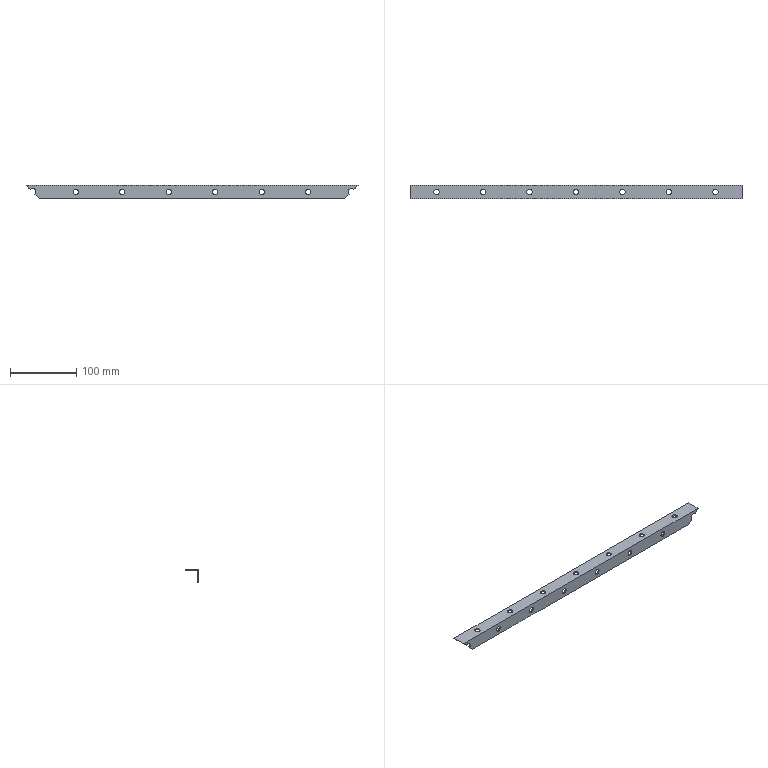Component | SolidWorks | AngleIron2-2 | 1 solid | 39 faces | box 500 x 20 x 20 mm | volume 35664 mm3 | cylinder 29 | plane 10 | commonest cylinder face diameters 8 x26 10 x3
build123d program:
from build123d import *

# Parameters (mm, degrees)
BOSS_EXTRUDE1_DEPTH = 500
CUT_EXTRUDE1_DEPTH  = 501.799
CUT_EXTRUDE2_DEPTH  = 501.799
SKETCH4_R           = 4
CUT_EXTRUDE3_DEPTH  = 501.799
LPATTERN1_COUNT     = 4
LPATTERN1_PITCH     = 70
LPATTERN1_COL_COUNT = 4
LPATTERN1_COL_PITCH = 70
SKETCH5_R           = 4
CUT_EXTRUDE4_DEPTH  = 501.799
LPATTERN2_COUNT     = 6
LPATTERN2_PITCH     = 70
SKETCH6_R           = 5
CUT_EXTRUDE5_DEPTH  = 501.799


with BuildPart() as part:
    # Sketch1 → Boss-Extrude1 (new body)
    with BuildSketch(Plane.XY):
        Polygon((0, 0), (20, 0), (20, -2), (2, -2), (2, -20), (0, -20), align=None)
    extrude(amount=BOSS_EXTRUDE1_DEPTH)

    # Sketch2 → Cut-Extrude1 (cut, through all)
    with BuildSketch(Plane(origin=(0, 0, 0), x_dir=(1, 0, 0), z_dir=(0, 1, 0))):
        Polygon((0, -500), (20, -500), (20, -480), align=None)
    extrude(amount=-CUT_EXTRUDE1_DEPTH, mode=Mode.SUBTRACT)

    # Sketch3 → Cut-Extrude2 (cut, through all)
    with BuildSketch(Plane(origin=(0, 0, 0), x_dir=(1, 0, 0), z_dir=(0, 1, 0))):
        Polygon((20, 0), (20, -20), (0, 0), align=None)
    extrude(amount=-CUT_EXTRUDE2_DEPTH, mode=Mode.SUBTRACT)

    # Sketch4 → Cut-Extrude3 (cut, through all)
    with BuildSketch(Plane.ZY):
        with Locations((250, -10)):
            Circle(SKETCH4_R)
    cut_extrude3 = extrude(amount=-CUT_EXTRUDE3_DEPTH, mode=Mode.SUBTRACT)

    # LPattern1: Cut-Extrude3 ×4
    with Locations(*[(0, 0, i * LPATTERN1_PITCH) for i in range(1, LPATTERN1_COUNT)]):
        add(cut_extrude3, mode=Mode.SUBTRACT)

    # LPattern1 col: Cut-Extrude3 ×4
    with Locations(*[(0, 0, -i * LPATTERN1_COL_PITCH) for i in range(1, LPATTERN1_COL_COUNT)]):
        add(cut_extrude3, mode=Mode.SUBTRACT)

    # Sketch5 → Cut-Extrude4 (cut, through all)
    with BuildSketch(Plane(origin=(0, 0, 0), x_dir=(1, 0, 0), z_dir=(0, 1, 0))):
        with Locations(Location((10, -425, 0), (0, 0, 270))):
            Circle(SKETCH5_R)
    cut_extrude4 = extrude(amount=-CUT_EXTRUDE4_DEPTH, mode=Mode.SUBTRACT)

    # LPattern2: Cut-Extrude4 ×6
    with Locations(*[(0, 0, -i * LPATTERN2_PITCH) for i in range(1, LPATTERN2_COUNT)]):
        add(cut_extrude4, mode=Mode.SUBTRACT)

    # Sketch6 → Cut-Extrude5 (cut, through all)
    with BuildSketch(Plane(origin=(0, 0, 0), x_dir=(1, 0, 0), z_dir=(0, 1, 0))):
        with Locations((10, -10)):
            Circle(SKETCH6_R)
        with Locations((10, -490)):
            Circle(SKETCH6_R)
    extrude(amount=-CUT_EXTRUDE5_DEPTH, mode=Mode.SUBTRACT)


solid = part.part

# Placed as in the assembly
solid = solid.moved(Location((566.241, -543.715, 1468.724), (180, -90, 0)))